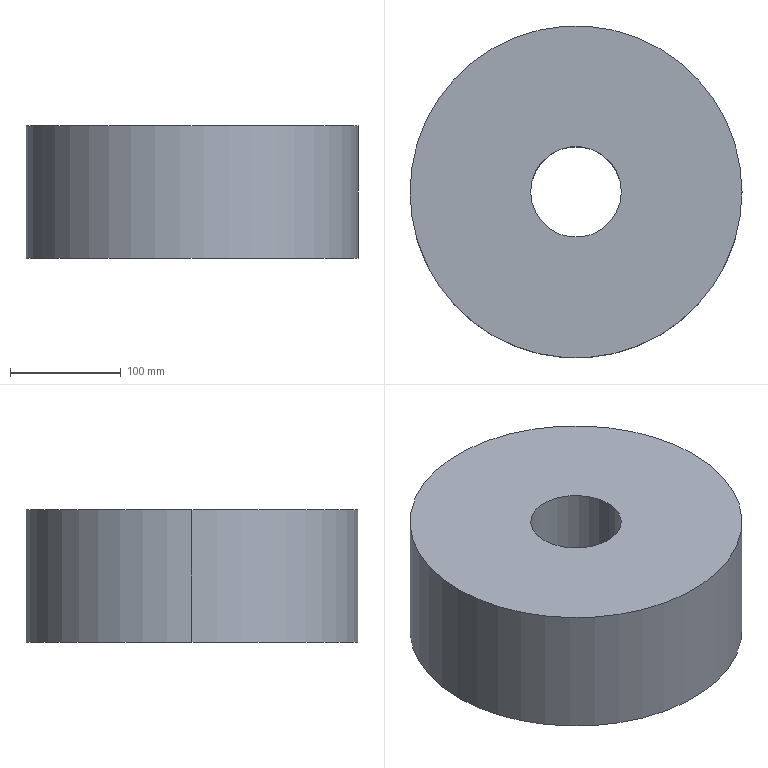Component | SolidWorks | MaximumCoilSize-1 | 1 solid | 6 faces | box 300 x 300 x 120 mm | volume 7848578 mm3 | cylinder 4 | plane 2 | commonest cylinder face diameters 82 x2 300 x2
build123d program:
from build123d import *

# Parameters (mm, degrees)
SKETCH1_R           = 150
SKETCH1_R_2         = 41
BOSS_EXTRUDE1_DEPTH = 60


with BuildPart() as part:
    # Sketch1 → Boss-Extrude1 (new, symmetric)
    with BuildSketch(Plane.XY):
        Circle(SKETCH1_R)
        Circle(SKETCH1_R_2, mode=Mode.SUBTRACT)
    extrude(amount=BOSS_EXTRUDE1_DEPTH, both=True)


solid = part.part

# Placed as in the assembly
solid = solid.moved(Location((733.029, 200.722, 172.5), (0, 0, 0)))
STEP:
#1=CARTESIAN_POINT('',(27.245,7.902,9.154));
#2=VERTEX_POINT('',#1);
#3=CARTESIAN_POINT('',(30.474,7.902,9.154));
#4=VERTEX_POINT('',#3);
#5=CARTESIAN_POINT('',(28.859,7.902,9.154));
#6=DIRECTION('',(0.,0.,1.));
#7=DIRECTION('',(1.,0.,0.));
#8=AXIS2_PLACEMENT_3D('',#5,#6,#7);
#9=CIRCLE('',#8,1.614);
#10=EDGE_CURVE('',#2,#4,#9,.T.);
#11=ORIENTED_EDGE('',*,*,#10,.T.);
#12=CARTESIAN_POINT('',(30.474,7.902,4.429));
#13=VERTEX_POINT('',#12);
#14=CARTESIAN_POINT('',(30.474,7.902,9.154));
#15=DIRECTION('',(0.,0.,-1.));
#16=VECTOR('',#15,39.37);
#17=LINE('',#14,#16);
#18=EDGE_CURVE('',#4,#13,#17,.T.);
#19=ORIENTED_EDGE('',*,*,#18,.T.);
#20=CARTESIAN_POINT('',(27.245,7.902,4.429));
#21=VERTEX_POINT('',#20);
#22=CARTESIAN_POINT('',(28.859,7.902,4.429));
#23=DIRECTION('',(0.,0.,1.));
#24=DIRECTION('',(1.,0.,0.));
#25=AXIS2_PLACEMENT_3D('',#22,#23,#24);
#26=CIRCLE('',#25,1.614);
#27=EDGE_CURVE('',#21,#13,#26,.T.);
#28=ORIENTED_EDGE('',*,*,#27,.F.);
#29=CARTESIAN_POINT('',(27.245,7.902,9.154));
#30=DIRECTION('',(0.,0.,-1.));
#31=VECTOR('',#30,39.37);
#32=LINE('',#29,#31);
#33=EDGE_CURVE('',#2,#21,#32,.T.);
#34=ORIENTED_EDGE('',*,*,#33,.F.);
#35=EDGE_LOOP('',(#11,#19,#28,#34));
#36=FACE_OUTER_BOUND('',#35,.T.);
#37=CARTESIAN_POINT('',(28.859,7.902,9.154));
#38=DIRECTION('',(0.,0.,-1.));
#39=DIRECTION('',(-1.,0.,0.));
#40=AXIS2_PLACEMENT_3D('',#37,#38,#39);
#41=CYLINDRICAL_SURFACE('',#40,1.614);
#42=ADVANCED_FACE('',(#36),#41,.F.);
#43=CARTESIAN_POINT('',(34.765,7.902,9.154));
#44=VERTEX_POINT('',#43);
#45=CARTESIAN_POINT('',(22.954,7.902,9.154));
#46=VERTEX_POINT('',#45);
#47=CARTESIAN_POINT('',(28.859,7.902,9.154));
#48=DIRECTION('',(0.,0.,1.));
#49=DIRECTION('',(1.,0.,0.));
#50=AXIS2_PLACEMENT_3D('',#47,#48,#49);
#51=CIRCLE('',#50,5.906);
#52=EDGE_CURVE('',#44,#46,#51,.T.);
#53=ORIENTED_EDGE('',*,*,#52,.F.);
#54=CARTESIAN_POINT('',(34.765,7.902,4.429));
#55=VERTEX_POINT('',#54);
#56=CARTESIAN_POINT('',(34.765,7.902,9.154));
#57=DIRECTION('',(0.,0.,-1.));
#58=VECTOR('',#57,39.37);
#59=LINE('',#56,#58);
#60=EDGE_CURVE('',#44,#55,#59,.T.);
#61=ORIENTED_EDGE('',*,*,#60,.T.);
#62=CARTESIAN_POINT('',(22.954,7.902,4.429));
#63=VERTEX_POINT('',#62);
#64=CARTESIAN_POINT('',(28.859,7.902,4.429));
#65=DIRECTION('',(0.,0.,1.));
#66=DIRECTION('',(1.,0.,0.));
#67=AXIS2_PLACEMENT_3D('',#64,#65,#66);
#68=CIRCLE('',#67,5.906);
#69=EDGE_CURVE('',#55,#63,#68,.T.);
#70=ORIENTED_EDGE('',*,*,#69,.T.);
#71=CARTESIAN_POINT('',(22.954,7.902,9.154));
#72=DIRECTION('',(0.,0.,-1.));
#73=VECTOR('',#72,39.37);
#74=LINE('',#71,#73);
#75=EDGE_CURVE('',#46,#63,#74,.T.);
#76=ORIENTED_EDGE('',*,*,#75,.F.);
#77=EDGE_LOOP('',(#53,#61,#70,#76));
#78=FACE_OUTER_BOUND('',#77,.T.);
#79=CARTESIAN_POINT('',(28.859,7.902,9.154));
#80=DIRECTION('',(0.,0.,-1.));
#81=DIRECTION('',(-1.,0.,0.));
#82=AXIS2_PLACEMENT_3D('',#79,#80,#81);
#83=CYLINDRICAL_SURFACE('',#82,5.906);
#84=ADVANCED_FACE('',(#78),#83,.T.);
#85=CARTESIAN_POINT('',(28.859,7.902,9.154));
#86=DIRECTION('',(0.,0.,1.));
#87=DIRECTION('',(1.,0.,0.));
#88=AXIS2_PLACEMENT_3D('',#85,#86,#87);
#89=CIRCLE('',#88,5.906);
#90=EDGE_CURVE('',#46,#44,#89,.T.);
#91=ORIENTED_EDGE('',*,*,#90,.T.);
#92=ORIENTED_EDGE('',*,*,#52,.T.);
#93=EDGE_LOOP('',(#91,#92));
#94=FACE_OUTER_BOUND('',#93,.T.);
#95=ORIENTED_EDGE('',*,*,#10,.F.);
#96=CARTESIAN_POINT('',(28.859,7.902,9.154));
#97=DIRECTION('',(0.,0.,1.));
#98=DIRECTION('',(1.,0.,0.));
#99=AXIS2_PLACEMENT_3D('',#96,#97,#98);
#100=CIRCLE('',#99,1.614);
#101=EDGE_CURVE('',#4,#2,#100,.T.);
#102=ORIENTED_EDGE('',*,*,#101,.F.);
#103=EDGE_LOOP('',(#95,#102));
#104=FACE_BOUND('',#103,.T.);
#105=CARTESIAN_POINT('',(28.859,7.902,9.154));
#106=DIRECTION('',(0.,0.,1.));
#107=DIRECTION('',(1.,0.,0.));
#108=AXIS2_PLACEMENT_3D('',#105,#106,#107);
#109=PLANE('',#108);
#110=ADVANCED_FACE('',(#94,#104),#109,.T.);
#111=CARTESIAN_POINT('',(28.859,7.902,4.429));
#112=DIRECTION('',(0.,0.,1.));
#113=DIRECTION('',(1.,0.,0.));
#114=AXIS2_PLACEMENT_3D('',#111,#112,#113);
#115=CIRCLE('',#114,5.906);
#116=EDGE_CURVE('',#63,#55,#115,.T.);
#117=ORIENTED_EDGE('',*,*,#116,.F.);
#118=ORIENTED_EDGE('',*,*,#69,.F.);
#119=EDGE_LOOP('',(#117,#118));
#120=FACE_OUTER_BOUND('',#119,.T.);
#121=ORIENTED_EDGE('',*,*,#27,.T.);
#122=CARTESIAN_POINT('',(28.859,7.902,4.429));
#123=DIRECTION('',(0.,0.,1.));
#124=DIRECTION('',(1.,0.,0.));
#125=AXIS2_PLACEMENT_3D('',#122,#123,#124);
#126=CIRCLE('',#125,1.614);
#127=EDGE_CURVE('',#13,#21,#126,.T.);
#128=ORIENTED_EDGE('',*,*,#127,.T.);
#129=EDGE_LOOP('',(#121,#128));
#130=FACE_BOUND('',#129,.T.);
#131=CARTESIAN_POINT('',(28.859,7.902,4.429));
#132=DIRECTION('',(0.,0.,1.));
#133=DIRECTION('',(1.,0.,0.));
#134=AXIS2_PLACEMENT_3D('',#131,#132,#133);
#135=PLANE('',#134);
#136=ADVANCED_FACE('',(#120,#130),#135,.F.);
#137=ORIENTED_EDGE('',*,*,#60,.F.);
#138=ORIENTED_EDGE('',*,*,#90,.F.);
#139=ORIENTED_EDGE('',*,*,#75,.T.);
#140=ORIENTED_EDGE('',*,*,#116,.T.);
#141=EDGE_LOOP('',(#137,#138,#139,#140));
#142=FACE_OUTER_BOUND('',#141,.T.);
#143=CARTESIAN_POINT('',(28.859,7.902,9.154));
#144=DIRECTION('',(0.,0.,-1.));
#145=DIRECTION('',(-1.,0.,0.));
#146=AXIS2_PLACEMENT_3D('',#143,#144,#145);
#147=CYLINDRICAL_SURFACE('',#146,5.906);
#148=ADVANCED_FACE('',(#142),#147,.T.);
#149=ORIENTED_EDGE('',*,*,#18,.F.);
#150=ORIENTED_EDGE('',*,*,#101,.T.);
#151=ORIENTED_EDGE('',*,*,#33,.T.);
#152=ORIENTED_EDGE('',*,*,#127,.F.);
#153=EDGE_LOOP('',(#149,#150,#151,#152));
#154=FACE_OUTER_BOUND('',#153,.T.);
#155=CARTESIAN_POINT('',(28.859,7.902,9.154));
#156=DIRECTION('',(0.,0.,-1.));
#157=DIRECTION('',(-1.,0.,0.));
#158=AXIS2_PLACEMENT_3D('',#155,#156,#157);
#159=CYLINDRICAL_SURFACE('',#158,1.614);
#160=ADVANCED_FACE('',(#154),#159,.F.);
#161=CLOSED_SHELL('',(#42,#84,#110,#136,#148,#160));
#162=MANIFOLD_SOLID_BREP('',#161);
#163=CARTESIAN_POINT('',(0.,0.,0.));
#164=DIRECTION('',(0.,0.,1.));
#165=DIRECTION('',(1.,0.,0.));
#166=AXIS2_PLACEMENT_3D('',#163,#164,#165);
#167=(LENGTH_UNIT()NAMED_UNIT(*)SI_UNIT($,.METRE.));
#168=LENGTH_MEASURE_WITH_UNIT(LENGTH_MEASURE(0.0254),#167);
#169=DIMENSIONAL_EXPONENTS(1.,0.,0.,0.,0.,0.,0.);
#170=(CONVERSION_BASED_UNIT('',#168)LENGTH_UNIT()NAMED_UNIT(#169));
#171=UNCERTAINTY_MEASURE_WITH_UNIT(LENGTH_MEASURE(0.00001),#170,'','');
#172=(NAMED_UNIT(*)PLANE_ANGLE_UNIT()SI_UNIT($,.RADIAN.));
#173=(NAMED_UNIT(*)SI_UNIT($,.STERADIAN.)SOLID_ANGLE_UNIT());
#174=(GEOMETRIC_REPRESENTATION_CONTEXT(3)GLOBAL_UNCERTAINTY_ASSIGNED_CONTEXT((#171))GLOBAL_UNIT_ASSIGNED_CONTEXT((#170,#172,#173))REPRESENTATION_CONTEXT('',''));
#175=ADVANCED_BREP_SHAPE_REPRESENTATION('',(#162,#166),#174);
#176=COLOUR_RGB('',0.7922,0.8196,0.9333);
#177=FILL_AREA_STYLE_COLOUR('',#176);
#178=FILL_AREA_STYLE('',(#177));
#179=SURFACE_STYLE_FILL_AREA(#178);
#180=SURFACE_SIDE_STYLE('',(#179));
#181=SURFACE_STYLE_USAGE(.BOTH.,#180);
#182=PRESENTATION_STYLE_ASSIGNMENT((#181));
#183=STYLED_ITEM('',(#182),#162);
#184=PRESENTATION_LAYER_ASSIGNMENT('','',(#183));
#185=(LENGTH_UNIT()NAMED_UNIT(*)SI_UNIT($,.METRE.));
#186=LENGTH_MEASURE_WITH_UNIT(LENGTH_MEASURE(0.0254),#185);
#187=DIMENSIONAL_EXPONENTS(1.,0.,0.,0.,0.,0.,0.);
#188=(CONVERSION_BASED_UNIT('',#186)LENGTH_UNIT()NAMED_UNIT(#187));
#189=UNCERTAINTY_MEASURE_WITH_UNIT(LENGTH_MEASURE(0.00001),#188,'','');
#190=(NAMED_UNIT(*)PLANE_ANGLE_UNIT()SI_UNIT($,.RADIAN.));
#191=(NAMED_UNIT(*)SI_UNIT($,.STERADIAN.)SOLID_ANGLE_UNIT());
#192=(GEOMETRIC_REPRESENTATION_CONTEXT(3)GLOBAL_UNCERTAINTY_ASSIGNED_CONTEXT((#189))GLOBAL_UNIT_ASSIGNED_CONTEXT((#188,#190,#191))REPRESENTATION_CONTEXT('',''));
#193=MECHANICAL_DESIGN_GEOMETRIC_PRESENTATION_REPRESENTATION('',(#183),#192);